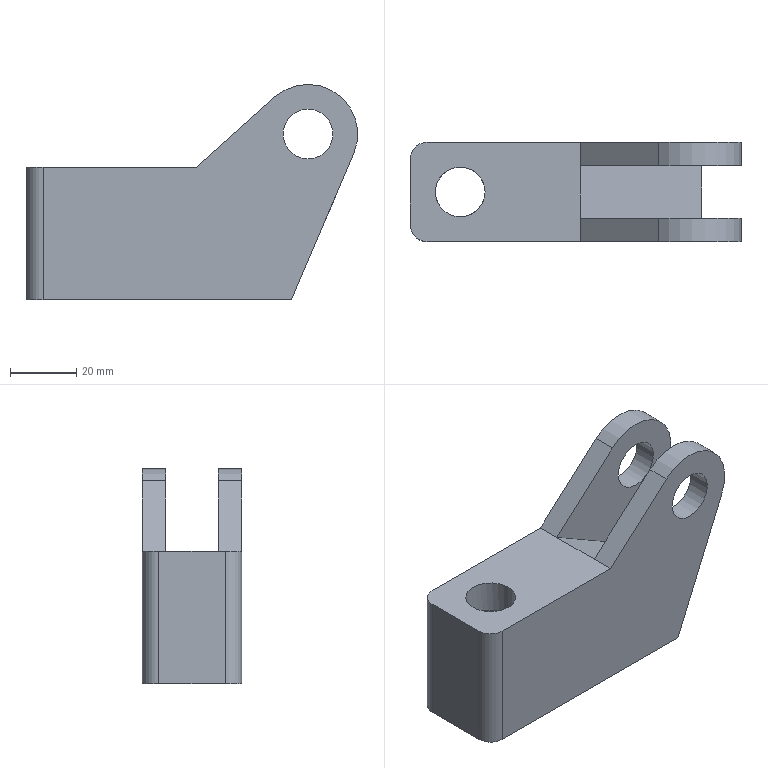Component | NX | UP_DOWN_BRACKET | 1 solid | 20 faces | volume 95628 mm3 | plane 12 | cylinder 8 | commonest cylinder face diameters 15 x3 30 x2 10 x2 20 x1